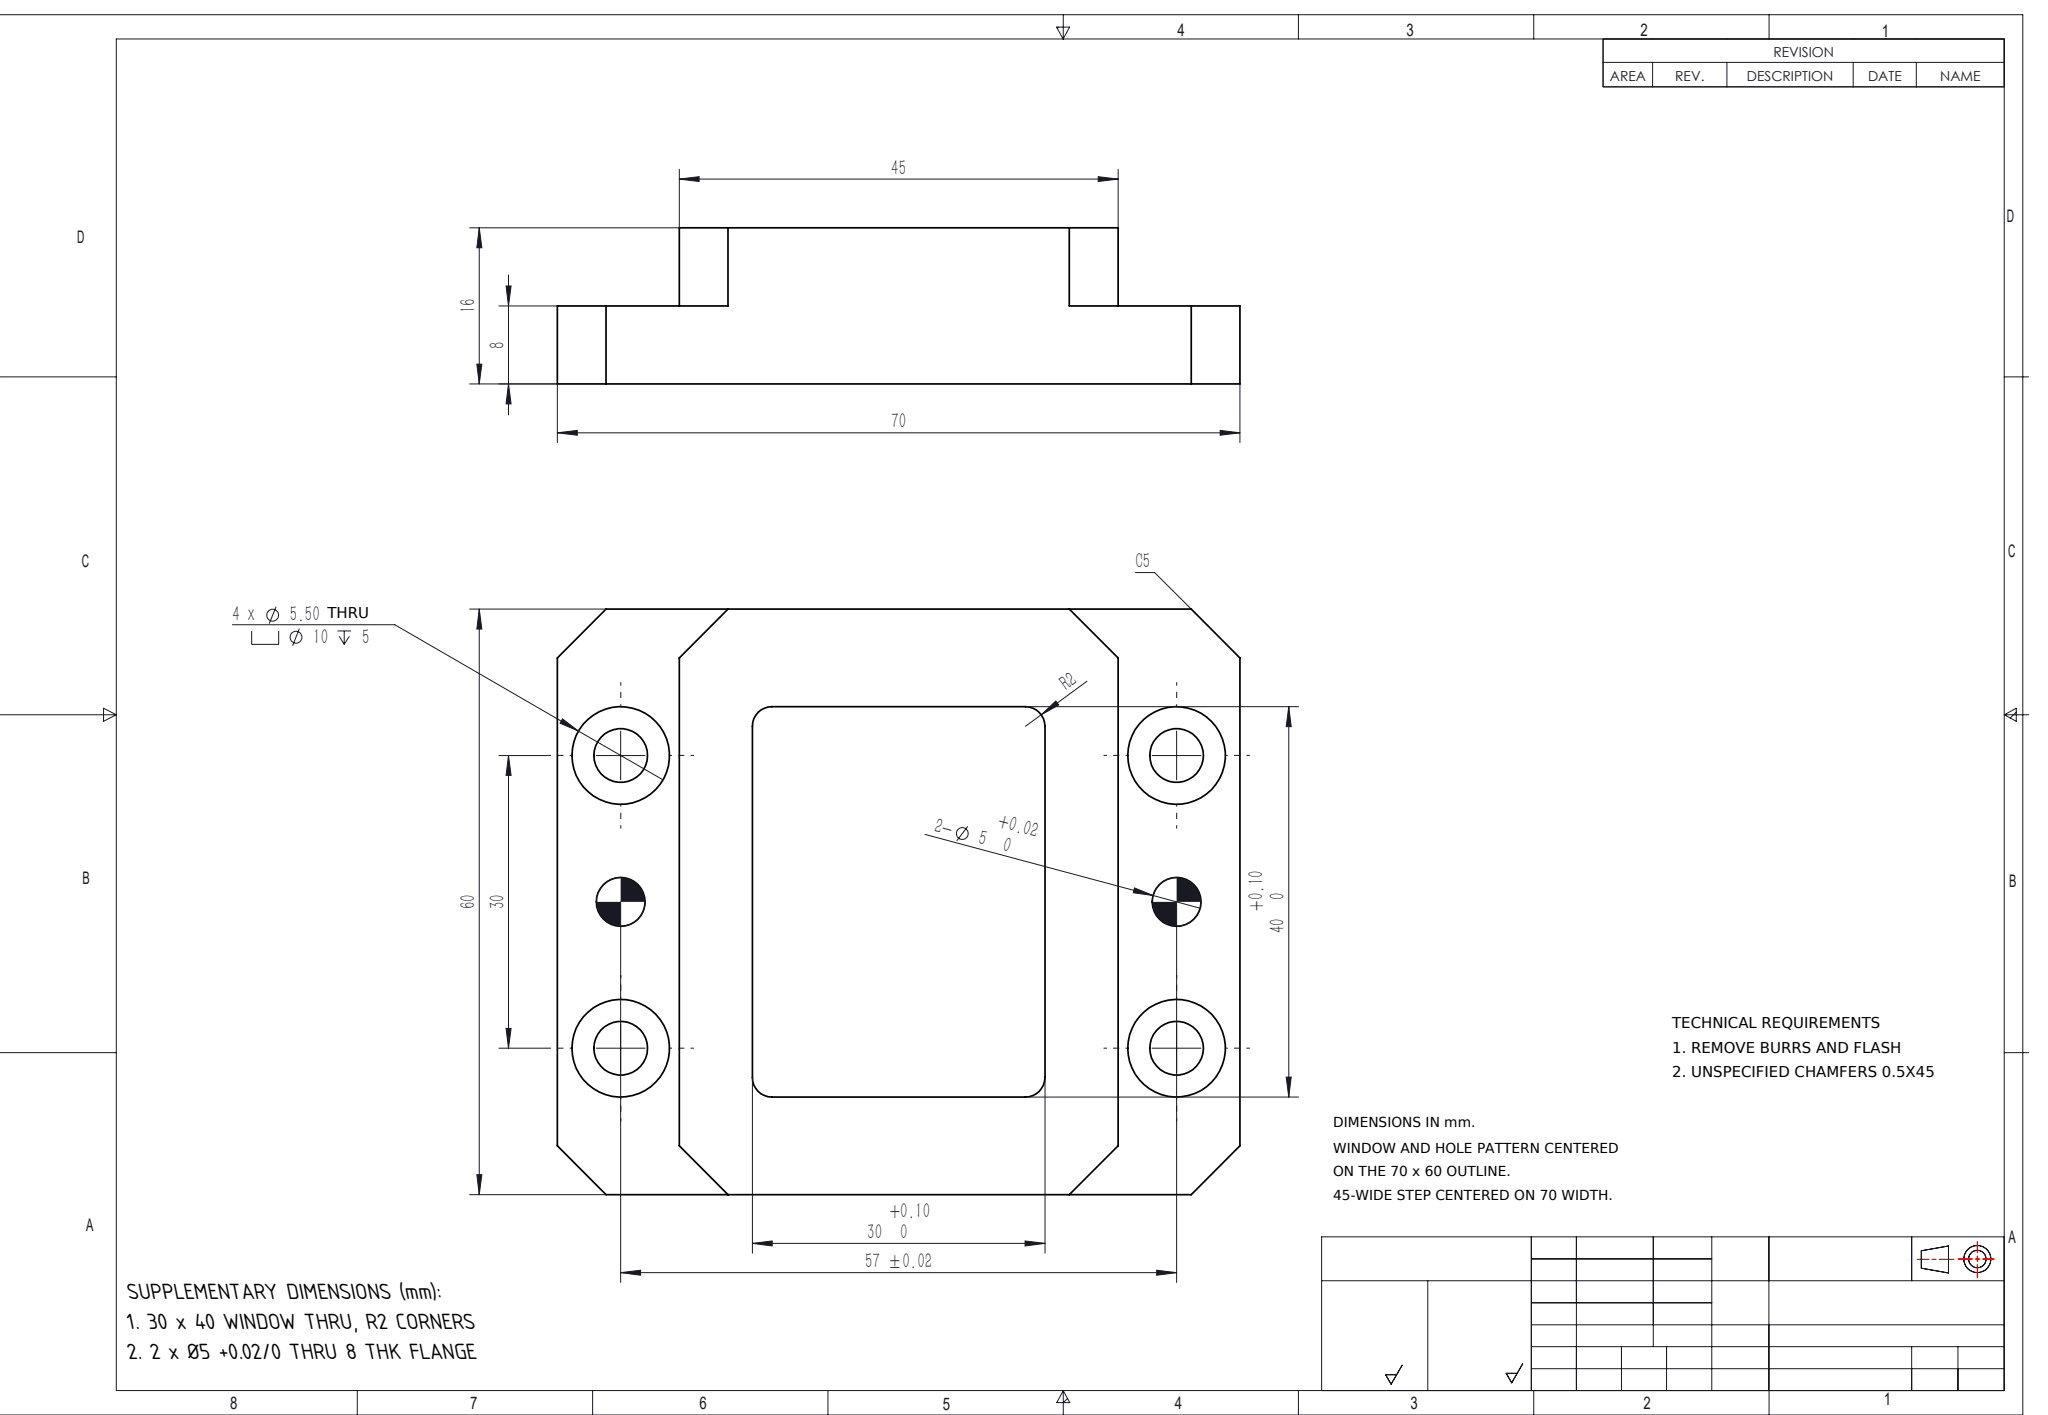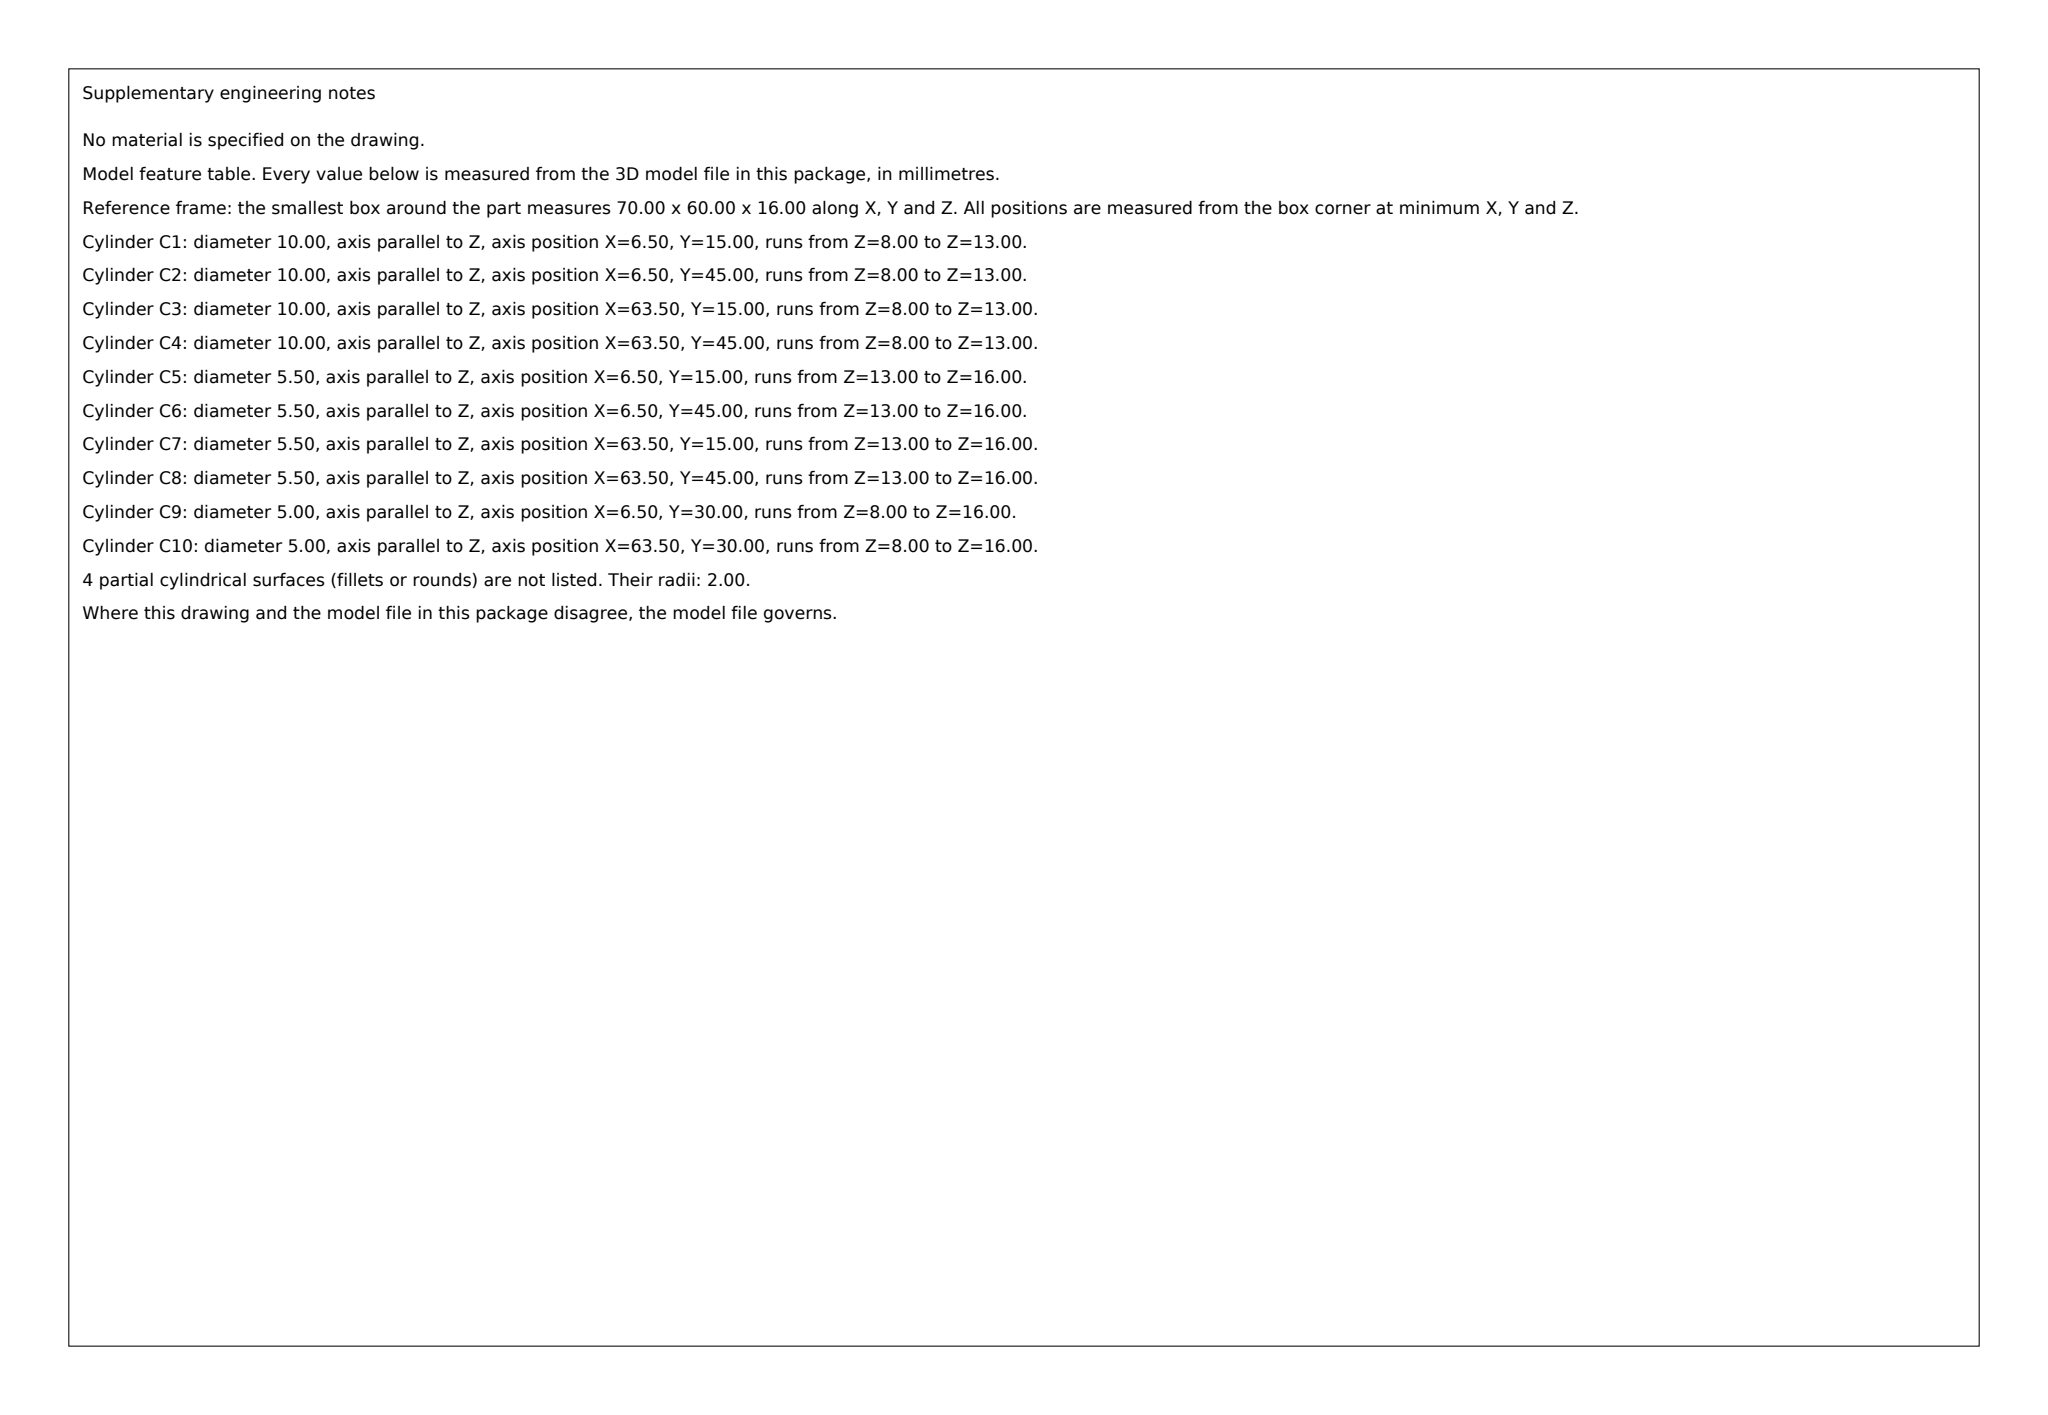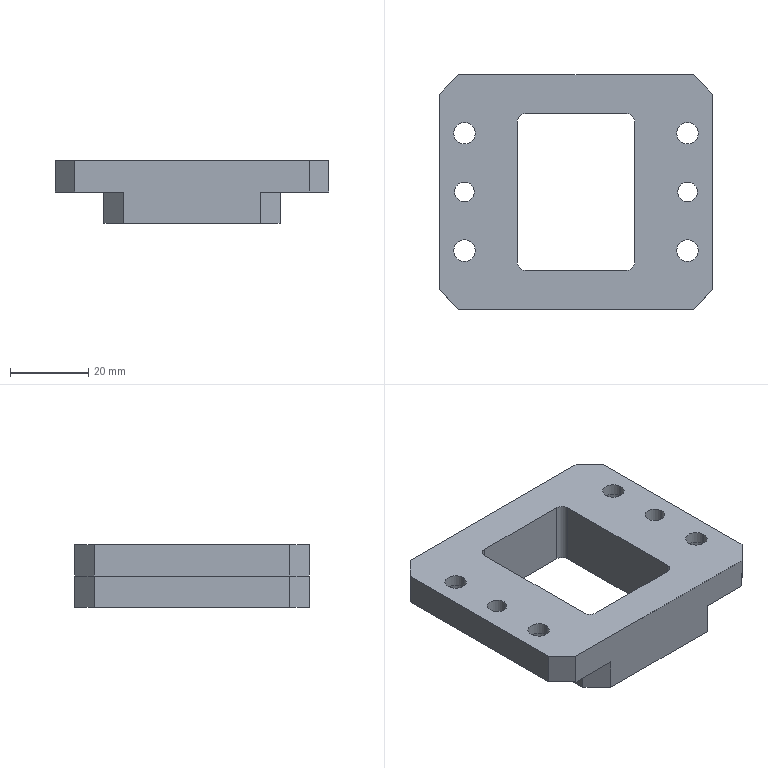Part | SolidWorks | mm | 1 solid | 50 faces | box 70 x 60 x 16 mm | volume 33085 mm3 | plane 26 | cylinder 24 | commonest cylinder face diameters 10 x8 5.5 x8 5 x4 4 x4
build123d program:
from build123d import *

# Parameters (mm, degrees)
SKETCH1_W                                       = 70
SKETCH1_H                                       = 60
BOSS_EXTRUDE1_DEPTH                             = 16
SKETCH2_W                                       = 12.5
SKETCH2_H                                       = 60
CUT_EXTRUDE1_DEPTH                              = 8
SKETCH3_W                                       = 30
SKETCH3_H                                       = 40
CUT_EXTRUDE2_DEPTH                              = 49.795
CHAMFER1_SIZE                                   = 5
CHAMFER2_SIZE                                   = 5
M5_HEX_SOCKET_HEAD_CAP_SCREW_CBORE1_D           = 5.5
M5_HEX_SOCKET_HEAD_CAP_SCREW_CBORE1_CBORE_D     = 10
M5_HEX_SOCKET_HEAD_CAP_SCREW_CBORE1_CBORE_DEPTH = 5
SIZE_MM_DOWEL_PIN_HOLE1_D                       = 5
FILLET1_R                                       = 2


with BuildPart() as part:
    # Sketch1 → Boss-Extrude1 (new body)
    with BuildSketch(Plane.XY):
        Rectangle(SKETCH1_W, SKETCH1_H)
    extrude(amount=BOSS_EXTRUDE1_DEPTH)

    # Sketch2 → Cut-Extrude1 (cut)
    with BuildSketch(Plane(origin=(0, 0, 0), x_dir=(-1, 0, 0), z_dir=(0, 0, -1))):
        with Locations((28.75, 0)):
            Rectangle(SKETCH2_W, SKETCH2_H)
        with Locations((-28.75, 0)):
            Rectangle(SKETCH2_W, SKETCH2_H)
    extrude(amount=-CUT_EXTRUDE1_DEPTH, mode=Mode.SUBTRACT)

    # Sketch3 → Cut-Extrude2 (cut, through all)
    with BuildSketch(Plane.XY.offset(16)):
        Rectangle(SKETCH3_W, SKETCH3_H)
    extrude(amount=-CUT_EXTRUDE2_DEPTH, mode=Mode.SUBTRACT)

    # Chamfer1
    chamfer1_edges = [part.edges().sort_by_distance(p)[0] for p in [
        (-22.5, -30, 4),
        (-22.5, 30, 4),
        (22.5, 30, 4),
        (22.5, -30, 4),
    ]]
    chamfer(chamfer1_edges, length=CHAMFER1_SIZE)

    # Chamfer2
    chamfer2_edges = [part.edges().sort_by_distance(p)[0] for p in [
        (35, -30, 12),
        (-35, -30, 12),
        (-35, 30, 12),
        (35, 30, 12),
    ]]
    chamfer(chamfer2_edges, length=CHAMFER2_SIZE)

    # M5 Hex Socket Head Cap Screw CBORE1 (through all)
    with Locations(Plane(origin=(0, 0, 8), x_dir=(1, 0, 0), z_dir=(0, 0, -1))):
        with Locations((28.5, 15), (28.5, -15), (-28.5, 15), (-28.5, -15)):
            CounterBoreHole(M5_HEX_SOCKET_HEAD_CAP_SCREW_CBORE1_D / 2, M5_HEX_SOCKET_HEAD_CAP_SCREW_CBORE1_CBORE_D / 2, M5_HEX_SOCKET_HEAD_CAP_SCREW_CBORE1_CBORE_DEPTH)

    # Size mm Dowel Pin Hole1 (through all)
    with Locations(Plane(origin=(0, 0, 8), x_dir=(-1, 0, 0), z_dir=(0, 0, -1))):
        with Locations((-28.5, 0), (28.5, 0)):
            Hole(SIZE_MM_DOWEL_PIN_HOLE1_D / 2)

    # Fillet1
    fillet1_edges = [part.edges().sort_by_distance(p)[0] for p in [
        (15, 20, 8),
        (15, -20, 8),
        (-15, -20, 8),
        (-15, 20, 8),
    ]]
    fillet(fillet1_edges, radius=FILLET1_R)


solid = part.part